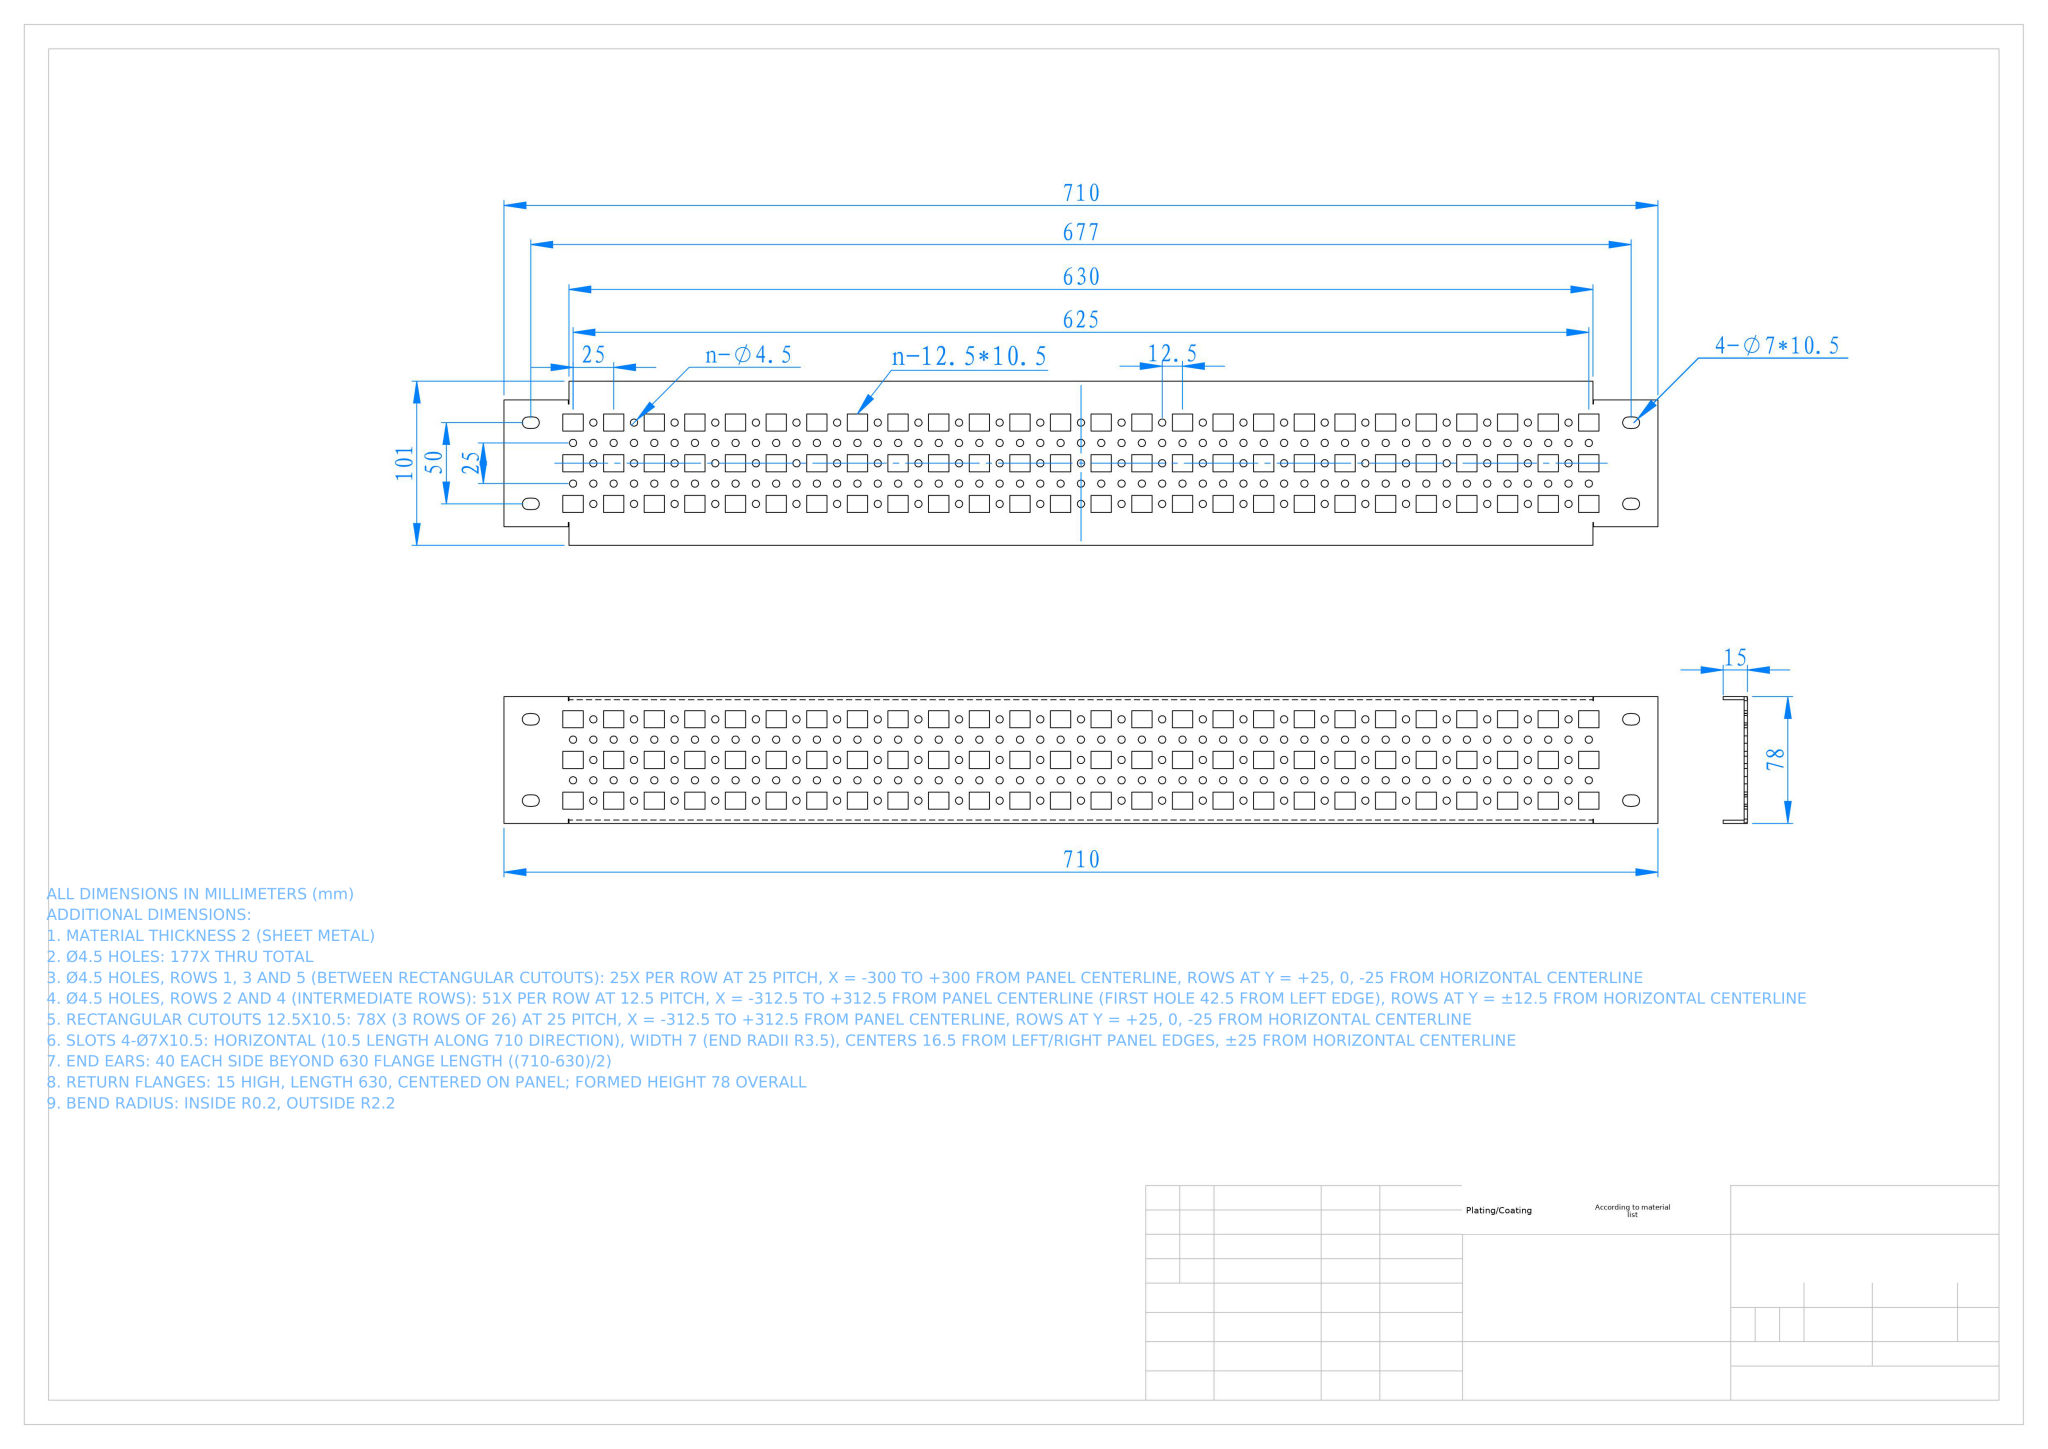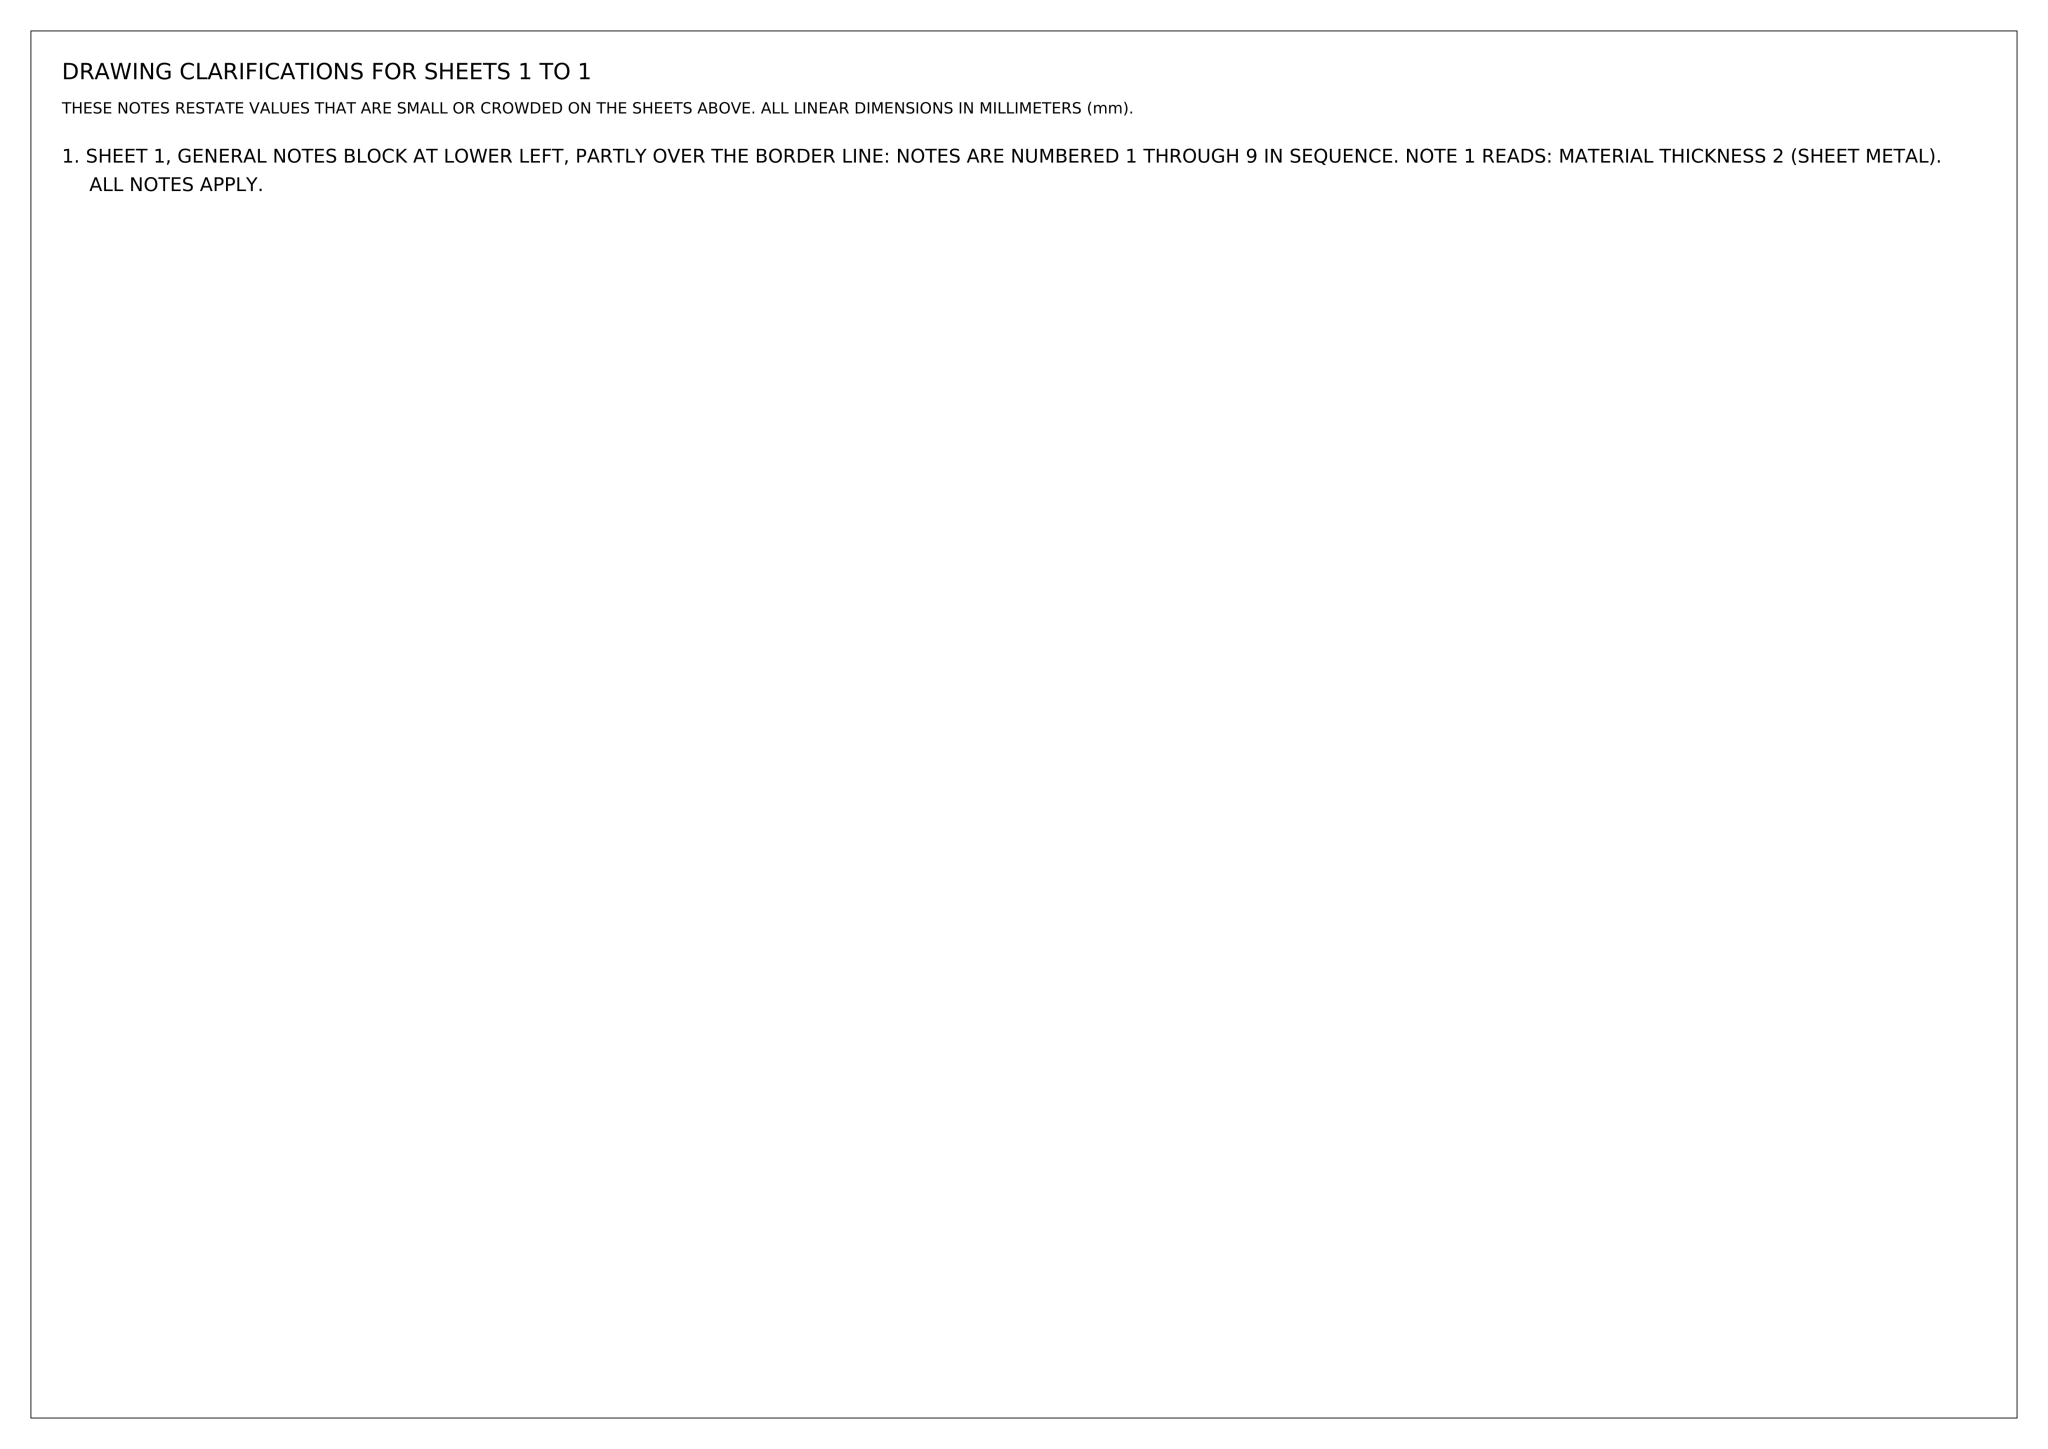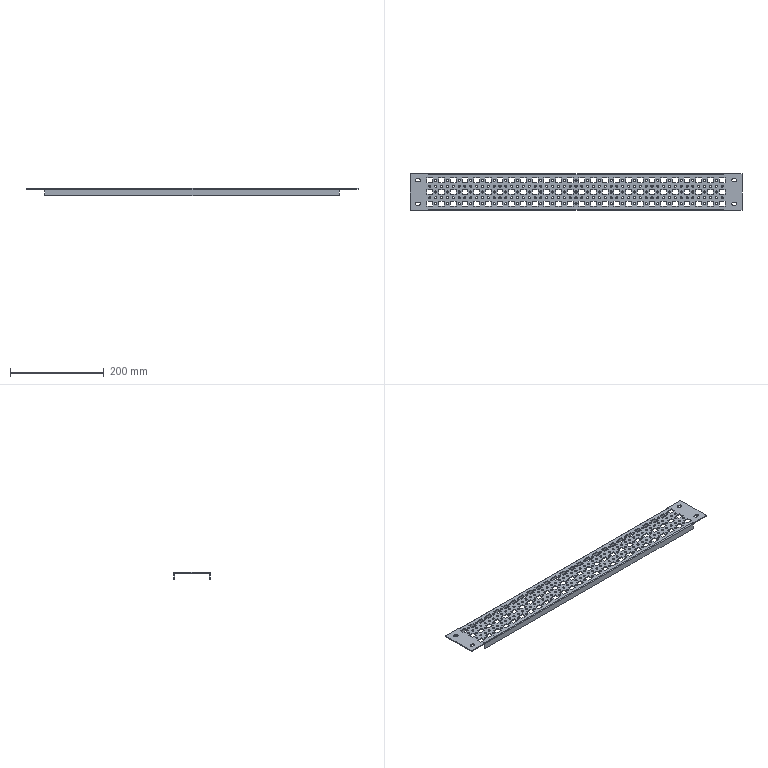Part | NX | mm | 1 solid | 740 faces | box 710 x 78 x 15 mm | volume 115603 mm3 | cylinder 378 | plane 362 | commonest cylinder face diameters 4.5 x354 7 x12 7.2 x8 4.4 x2 0.4 x2